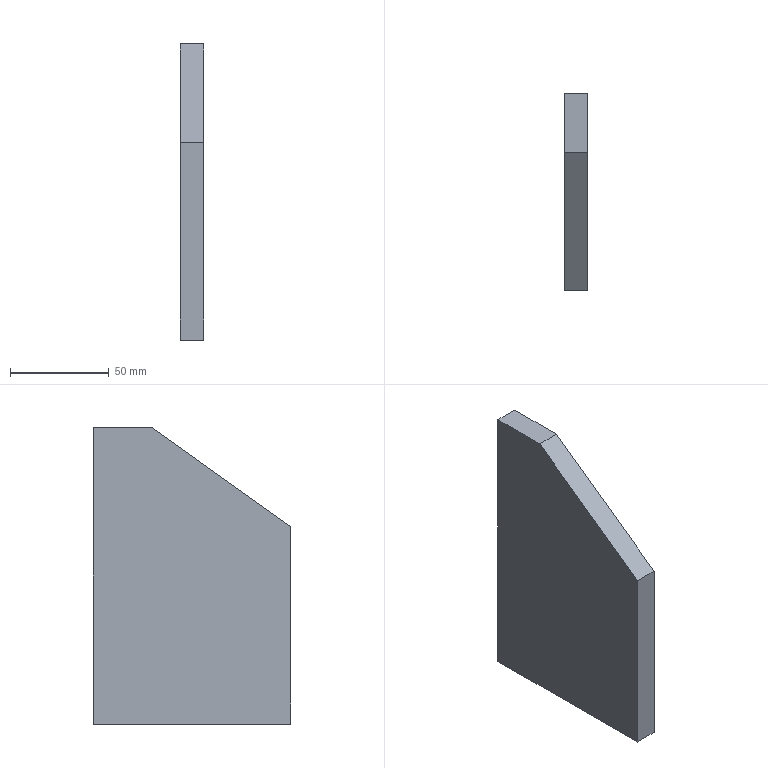Component | SolidWorks | 8TC-A15004-80-04A-1 | 1 solid | 27 faces | box 12 x 100 x 150 mm | volume 156512 mm3 | cylinder 10 | cone 10 | plane 7 | commonest cylinder face diameters 6 x10 | material A3
build123d program:
from build123d import *

# Parameters (mm, degrees)
BOSS_EXTRUDE1_DEPTH   = 6
M6_TAPPED_HOLE1_D     = 6
M6_TAPPED_HOLE1_DEPTH = 17
M6_TAPPED_HOLE1_TIP   = 1.803
M6_TAPPED_HOLE2_D     = 6
M6_TAPPED_HOLE2_DEPTH = 17
M6_TAPPED_HOLE2_TIP   = 1.803


with BuildPart() as part:
    # Sketch1 → Boss-Extrude1 (new, symmetric)
    with BuildSketch(Plane(origin=(0, 0, 0), x_dir=(1, 0, 0), z_dir=(0, 1, 0))):
        Polygon((0, 0), (0, 150), (30, 150), (100, 100), (100, 0), align=None)
    extrude(amount=BOSS_EXTRUDE1_DEPTH, both=True)

    # M6 Tapped Hole1
    with Locations(Plane.ZY):
        with Locations((-30, 0), (-80, 0), (-130, 0)):
            Hole(M6_TAPPED_HOLE1_D / 2, depth=M6_TAPPED_HOLE1_DEPTH)
            with Locations((0, 0, -(M6_TAPPED_HOLE1_DEPTH + M6_TAPPED_HOLE1_TIP / 2))):  # 118° drill point
                Cone(0, M6_TAPPED_HOLE1_D / 2, M6_TAPPED_HOLE1_TIP, mode=Mode.SUBTRACT)

    # M6 Tapped Hole2
    with Locations(Plane.XY):
        with Locations((20, 0), (80, 0)):
            Hole(M6_TAPPED_HOLE2_D / 2, depth=M6_TAPPED_HOLE2_DEPTH)
            with Locations((0, 0, -(M6_TAPPED_HOLE2_DEPTH + M6_TAPPED_HOLE2_TIP / 2))):  # 118° drill point
                Cone(0, M6_TAPPED_HOLE2_D / 2, M6_TAPPED_HOLE2_TIP, mode=Mode.SUBTRACT)


solid = part.part

# Placed as in the assembly
solid = solid.moved(Location((16, -7.5, 40), (180, 0, 90)))
STEP:
#1=COLOUR_RGB('',0.7922,0.8196,0.9333);
#2=FILL_AREA_STYLE_COLOUR('',#1);
#3=FILL_AREA_STYLE('',(#2));
#4=SURFACE_STYLE_FILL_AREA(#3);
#5=SURFACE_SIDE_STYLE('',(#4));
#6=SURFACE_STYLE_USAGE(.BOTH.,#5);
#7=PRESENTATION_STYLE_ASSIGNMENT((#6));
#8=CARTESIAN_POINT('',(0.6299,-0.9646,2.244));
#9=VERTEX_POINT('',#8);
#10=CARTESIAN_POINT('',(0.6299,-1.201,2.244));
#11=VERTEX_POINT('',#10);
#12=CARTESIAN_POINT('',(0.6299,-1.083,2.244));
#13=DIRECTION('',(0.,0.,-1.));
#14=DIRECTION('',(0.,-1.,0.));
#15=AXIS2_PLACEMENT_3D('',#12,#13,#14);
#16=CIRCLE('',#15,0.1181);
#17=EDGE_CURVE('',#9,#11,#16,.T.);
#18=ORIENTED_EDGE('',*,*,#17,.F.);
#19=CARTESIAN_POINT('',(0.6299,-0.9646,1.575));
#20=VERTEX_POINT('',#19);
#21=CARTESIAN_POINT('',(0.6299,-0.9646,1.575));
#22=DIRECTION('',(0.,0.,-1.));
#23=VECTOR('',#22,39.37);
#24=LINE('',#21,#23);
#25=EDGE_CURVE('',#9,#20,#24,.T.);
#26=ORIENTED_EDGE('',*,*,#25,.T.);
#27=CARTESIAN_POINT('',(0.6299,-1.201,1.575));
#28=VERTEX_POINT('',#27);
#29=CARTESIAN_POINT('',(0.6299,-1.083,1.575));
#30=DIRECTION('',(0.,0.,-1.));
#31=DIRECTION('',(0.,-1.,0.));
#32=AXIS2_PLACEMENT_3D('',#29,#30,#31);
#33=CIRCLE('',#32,0.1181);
#34=EDGE_CURVE('',#20,#28,#33,.T.);
#35=ORIENTED_EDGE('',*,*,#34,.T.);
#36=CARTESIAN_POINT('',(0.6299,-1.201,1.575));
#37=DIRECTION('',(0.,0.,-1.));
#38=VECTOR('',#37,39.37);
#39=LINE('',#36,#38);
#40=EDGE_CURVE('',#11,#28,#39,.T.);
#41=ORIENTED_EDGE('',*,*,#40,.F.);
#42=EDGE_LOOP('',(#18,#26,#35,#41));
#43=FACE_OUTER_BOUND('',#42,.T.);
#44=CARTESIAN_POINT('',(0.6299,-1.083,1.575));
#45=DIRECTION('',(0.,0.,-1.));
#46=DIRECTION('',(0.,-1.,0.));
#47=AXIS2_PLACEMENT_3D('',#44,#45,#46);
#48=CYLINDRICAL_SURFACE('',#47,0.1181);
#49=ADVANCED_FACE('',(#43),#48,.F.);
#50=CARTESIAN_POINT('',(0.6299,-1.083,2.315));
#51=VERTEX_POINT('',#50);
#52=CARTESIAN_POINT('',(0.6299,-1.201,2.244));
#53=DIRECTION('',(0.,-0.8572,-0.515));
#54=VECTOR('',#53,39.37);
#55=LINE('',#52,#54);
#56=EDGE_CURVE('',#51,#11,#55,.T.);
#57=ORIENTED_EDGE('',*,*,#56,.F.);
#58=CARTESIAN_POINT('',(0.6299,-0.9646,2.244));
#59=DIRECTION('',(-0.,0.8572,-0.515));
#60=VECTOR('',#59,39.37);
#61=LINE('',#58,#60);
#62=EDGE_CURVE('',#51,#9,#61,.T.);
#63=ORIENTED_EDGE('',*,*,#62,.T.);
#64=ORIENTED_EDGE('',*,*,#17,.T.);
#65=EDGE_LOOP('',(#57,#63,#64));
#66=FACE_OUTER_BOUND('',#65,.T.);
#67=CARTESIAN_POINT('',(0.6299,-1.083,2.244));
#68=DIRECTION('',(0.,0.,-1.));
#69=DIRECTION('',(0.,-1.,0.));
#70=AXIS2_PLACEMENT_3D('',#67,#68,#69);
#71=CONICAL_SURFACE('',#70,0.1181,1.03);
#72=ADVANCED_FACE('',(#66),#71,.F.);
#73=CARTESIAN_POINT('',(0.6299,-3.327,2.244));
#74=VERTEX_POINT('',#73);
#75=CARTESIAN_POINT('',(0.6299,-3.563,2.244));
#76=VERTEX_POINT('',#75);
#77=CARTESIAN_POINT('',(0.6299,-3.445,2.244));
#78=DIRECTION('',(0.,0.,-1.));
#79=DIRECTION('',(0.,-1.,0.));
#80=AXIS2_PLACEMENT_3D('',#77,#78,#79);
#81=CIRCLE('',#80,0.1181);
#82=EDGE_CURVE('',#74,#76,#81,.T.);
#83=ORIENTED_EDGE('',*,*,#82,.F.);
#84=CARTESIAN_POINT('',(0.6299,-3.327,1.575));
#85=VERTEX_POINT('',#84);
#86=CARTESIAN_POINT('',(0.6299,-3.327,1.575));
#87=DIRECTION('',(0.,0.,-1.));
#88=VECTOR('',#87,39.37);
#89=LINE('',#86,#88);
#90=EDGE_CURVE('',#74,#85,#89,.T.);
#91=ORIENTED_EDGE('',*,*,#90,.T.);
#92=CARTESIAN_POINT('',(0.6299,-3.563,1.575));
#93=VERTEX_POINT('',#92);
#94=CARTESIAN_POINT('',(0.6299,-3.445,1.575));
#95=DIRECTION('',(0.,0.,-1.));
#96=DIRECTION('',(0.,-1.,0.));
#97=AXIS2_PLACEMENT_3D('',#94,#95,#96);
#98=CIRCLE('',#97,0.1181);
#99=EDGE_CURVE('',#85,#93,#98,.T.);
#100=ORIENTED_EDGE('',*,*,#99,.T.);
#101=CARTESIAN_POINT('',(0.6299,-3.563,1.575));
#102=DIRECTION('',(0.,0.,-1.));
#103=VECTOR('',#102,39.37);
#104=LINE('',#101,#103);
#105=EDGE_CURVE('',#76,#93,#104,.T.);
#106=ORIENTED_EDGE('',*,*,#105,.F.);
#107=EDGE_LOOP('',(#83,#91,#100,#106));
#108=FACE_OUTER_BOUND('',#107,.T.);
#109=CARTESIAN_POINT('',(0.6299,-3.445,1.575));
#110=DIRECTION('',(0.,0.,-1.));
#111=DIRECTION('',(0.,-1.,0.));
#112=AXIS2_PLACEMENT_3D('',#109,#110,#111);
#113=CYLINDRICAL_SURFACE('',#112,0.1181);
#114=ADVANCED_FACE('',(#108),#113,.F.);
#115=CARTESIAN_POINT('',(0.6299,-3.445,2.315));
#116=VERTEX_POINT('',#115);
#117=CARTESIAN_POINT('',(0.6299,-3.563,2.244));
#118=DIRECTION('',(0.,-0.8572,-0.515));
#119=VECTOR('',#118,39.37);
#120=LINE('',#117,#119);
#121=EDGE_CURVE('',#116,#76,#120,.T.);
#122=ORIENTED_EDGE('',*,*,#121,.F.);
#123=CARTESIAN_POINT('',(0.6299,-3.327,2.244));
#124=DIRECTION('',(-0.,0.8572,-0.515));
#125=VECTOR('',#124,39.37);
#126=LINE('',#123,#125);
#127=EDGE_CURVE('',#116,#74,#126,.T.);
#128=ORIENTED_EDGE('',*,*,#127,.T.);
#129=ORIENTED_EDGE('',*,*,#82,.T.);
#130=EDGE_LOOP('',(#122,#128,#129));
#131=FACE_OUTER_BOUND('',#130,.T.);
#132=CARTESIAN_POINT('',(0.6299,-3.445,2.244));
#133=DIRECTION('',(0.,0.,-1.));
#134=DIRECTION('',(0.,-1.,0.));
#135=AXIS2_PLACEMENT_3D('',#132,#133,#134);
#136=CONICAL_SURFACE('',#135,0.1181,1.03);
#137=ADVANCED_FACE('',(#131),#136,.F.);
#138=CARTESIAN_POINT('',(0.6299,-0.9646,2.874));
#139=VERTEX_POINT('',#138);
#140=CARTESIAN_POINT('',(0.6299,-0.9646,2.638));
#141=VERTEX_POINT('',#140);
#142=CARTESIAN_POINT('',(0.6299,-0.9646,2.756));
#143=DIRECTION('',(-0.,1.,0.));
#144=DIRECTION('',(0.,0.,-1.));
#145=AXIS2_PLACEMENT_3D('',#142,#143,#144);
#146=CIRCLE('',#145,0.1181);
#147=EDGE_CURVE('',#139,#141,#146,.T.);
#148=ORIENTED_EDGE('',*,*,#147,.F.);
#149=CARTESIAN_POINT('',(0.6299,-0.2953,2.874));
#150=VERTEX_POINT('',#149);
#151=CARTESIAN_POINT('',(0.6299,-0.2953,2.874));
#152=DIRECTION('',(-0.,1.,0.));
#153=VECTOR('',#152,39.37);
#154=LINE('',#151,#153);
#155=EDGE_CURVE('',#139,#150,#154,.T.);
#156=ORIENTED_EDGE('',*,*,#155,.T.);
#157=CARTESIAN_POINT('',(0.6299,-0.2953,2.638));
#158=VERTEX_POINT('',#157);
#159=CARTESIAN_POINT('',(0.6299,-0.2953,2.756));
#160=DIRECTION('',(-0.,1.,0.));
#161=DIRECTION('',(0.,0.,-1.));
#162=AXIS2_PLACEMENT_3D('',#159,#160,#161);
#163=CIRCLE('',#162,0.1181);
#164=EDGE_CURVE('',#150,#158,#163,.T.);
#165=ORIENTED_EDGE('',*,*,#164,.T.);
#166=CARTESIAN_POINT('',(0.6299,-0.2953,2.638));
#167=DIRECTION('',(-0.,1.,0.));
#168=VECTOR('',#167,39.37);
#169=LINE('',#166,#168);
#170=EDGE_CURVE('',#141,#158,#169,.T.);
#171=ORIENTED_EDGE('',*,*,#170,.F.);
#172=EDGE_LOOP('',(#148,#156,#165,#171));
#173=FACE_OUTER_BOUND('',#172,.T.);
#174=CARTESIAN_POINT('',(0.6299,-0.2953,2.756));
#175=DIRECTION('',(-0.,1.,0.));
#176=DIRECTION('',(0.,0.,-1.));
#177=AXIS2_PLACEMENT_3D('',#174,#175,#176);
#178=CYLINDRICAL_SURFACE('',#177,0.1181);
#179=ADVANCED_FACE('',(#173),#178,.F.);
#180=CARTESIAN_POINT('',(0.6299,-1.036,2.756));
#181=VERTEX_POINT('',#180);
#182=CARTESIAN_POINT('',(0.6299,-0.9646,2.638));
#183=DIRECTION('',(-0.,0.515,-0.8572));
#184=VECTOR('',#183,39.37);
#185=LINE('',#182,#184);
#186=EDGE_CURVE('',#181,#141,#185,.T.);
#187=ORIENTED_EDGE('',*,*,#186,.F.);
#188=CARTESIAN_POINT('',(0.6299,-0.9646,2.874));
#189=DIRECTION('',(-0.,0.515,0.8572));
#190=VECTOR('',#189,39.37);
#191=LINE('',#188,#190);
#192=EDGE_CURVE('',#181,#139,#191,.T.);
#193=ORIENTED_EDGE('',*,*,#192,.T.);
#194=ORIENTED_EDGE('',*,*,#147,.T.);
#195=EDGE_LOOP('',(#187,#193,#194));
#196=FACE_OUTER_BOUND('',#195,.T.);
#197=CARTESIAN_POINT('',(0.6299,-0.9646,2.756));
#198=DIRECTION('',(-0.,1.,0.));
#199=DIRECTION('',(0.,0.,-1.));
#200=AXIS2_PLACEMENT_3D('',#197,#198,#199);
#201=CONICAL_SURFACE('',#200,0.1181,1.03);
#202=ADVANCED_FACE('',(#196),#201,.F.);
#203=CARTESIAN_POINT('',(0.6299,-0.9646,4.843));
#204=VERTEX_POINT('',#203);
#205=CARTESIAN_POINT('',(0.6299,-0.9646,4.606));
#206=VERTEX_POINT('',#205);
#207=CARTESIAN_POINT('',(0.6299,-0.9646,4.724));
#208=DIRECTION('',(-0.,1.,0.));
#209=DIRECTION('',(0.,0.,-1.));
#210=AXIS2_PLACEMENT_3D('',#207,#208,#209);
#211=CIRCLE('',#210,0.1181);
#212=EDGE_CURVE('',#204,#206,#211,.T.);
#213=ORIENTED_EDGE('',*,*,#212,.F.);
#214=CARTESIAN_POINT('',(0.6299,-0.2953,4.843));
#215=VERTEX_POINT('',#214);
#216=CARTESIAN_POINT('',(0.6299,-0.2953,4.843));
#217=DIRECTION('',(-0.,1.,0.));
#218=VECTOR('',#217,39.37);
#219=LINE('',#216,#218);
#220=EDGE_CURVE('',#204,#215,#219,.T.);
#221=ORIENTED_EDGE('',*,*,#220,.T.);
#222=CARTESIAN_POINT('',(0.6299,-0.2953,4.606));
#223=VERTEX_POINT('',#222);
#224=CARTESIAN_POINT('',(0.6299,-0.2953,4.724));
#225=DIRECTION('',(-0.,1.,0.));
#226=DIRECTION('',(0.,0.,-1.));
#227=AXIS2_PLACEMENT_3D('',#224,#225,#226);
#228=CIRCLE('',#227,0.1181);
#229=EDGE_CURVE('',#215,#223,#228,.T.);
#230=ORIENTED_EDGE('',*,*,#229,.T.);
#231=CARTESIAN_POINT('',(0.6299,-0.2953,4.606));
#232=DIRECTION('',(-0.,1.,0.));
#233=VECTOR('',#232,39.37);
#234=LINE('',#231,#233);
#235=EDGE_CURVE('',#206,#223,#234,.T.);
#236=ORIENTED_EDGE('',*,*,#235,.F.);
#237=EDGE_LOOP('',(#213,#221,#230,#236));
#238=FACE_OUTER_BOUND('',#237,.T.);
#239=CARTESIAN_POINT('',(0.6299,-0.2953,4.724));
#240=DIRECTION('',(-0.,1.,0.));
#241=DIRECTION('',(0.,0.,-1.));
#242=AXIS2_PLACEMENT_3D('',#239,#240,#241);
#243=CYLINDRICAL_SURFACE('',#242,0.1181);
#244=ADVANCED_FACE('',(#238),#243,.F.);
#245=CARTESIAN_POINT('',(0.6299,-1.036,4.724));
#246=VERTEX_POINT('',#245);
#247=CARTESIAN_POINT('',(0.6299,-0.9646,4.606));
#248=DIRECTION('',(-0.,0.515,-0.8572));
#249=VECTOR('',#248,39.37);
#250=LINE('',#247,#249);
#251=EDGE_CURVE('',#246,#206,#250,.T.);
#252=ORIENTED_EDGE('',*,*,#251,.F.);
#253=CARTESIAN_POINT('',(0.6299,-0.9646,4.843));
#254=DIRECTION('',(-0.,0.515,0.8572));
#255=VECTOR('',#254,39.37);
#256=LINE('',#253,#255);
#257=EDGE_CURVE('',#246,#204,#256,.T.);
#258=ORIENTED_EDGE('',*,*,#257,.T.);
#259=ORIENTED_EDGE('',*,*,#212,.T.);
#260=EDGE_LOOP('',(#252,#258,#259));
#261=FACE_OUTER_BOUND('',#260,.T.);
#262=CARTESIAN_POINT('',(0.6299,-0.9646,4.724));
#263=DIRECTION('',(-0.,1.,0.));
#264=DIRECTION('',(0.,0.,-1.));
#265=AXIS2_PLACEMENT_3D('',#262,#263,#264);
#266=CONICAL_SURFACE('',#265,0.1181,1.03);
#267=ADVANCED_FACE('',(#261),#266,.F.);
#268=CARTESIAN_POINT('',(0.6299,-0.9646,6.811));
#269=VERTEX_POINT('',#268);
#270=CARTESIAN_POINT('',(0.6299,-0.9646,6.575));
#271=VERTEX_POINT('',#270);
#272=CARTESIAN_POINT('',(0.6299,-0.9646,6.693));
#273=DIRECTION('',(-0.,1.,0.));
#274=DIRECTION('',(0.,0.,-1.));
#275=AXIS2_PLACEMENT_3D('',#272,#273,#274);
#276=CIRCLE('',#275,0.1181);
#277=EDGE_CURVE('',#269,#271,#276,.T.);
#278=ORIENTED_EDGE('',*,*,#277,.F.);
#279=CARTESIAN_POINT('',(0.6299,-0.2953,6.811));
#280=VERTEX_POINT('',#279);
#281=CARTESIAN_POINT('',(0.6299,-0.2953,6.811));
#282=DIRECTION('',(-0.,1.,0.));
#283=VECTOR('',#282,39.37);
#284=LINE('',#281,#283);
#285=EDGE_CURVE('',#269,#280,#284,.T.);
#286=ORIENTED_EDGE('',*,*,#285,.T.);
#287=CARTESIAN_POINT('',(0.6299,-0.2953,6.575));
#288=VERTEX_POINT('',#287);
#289=CARTESIAN_POINT('',(0.6299,-0.2953,6.693));
#290=DIRECTION('',(-0.,1.,0.));
#291=DIRECTION('',(0.,0.,-1.));
#292=AXIS2_PLACEMENT_3D('',#289,#290,#291);
#293=CIRCLE('',#292,0.1181);
#294=EDGE_CURVE('',#280,#288,#293,.T.);
#295=ORIENTED_EDGE('',*,*,#294,.T.);
#296=CARTESIAN_POINT('',(0.6299,-0.2953,6.575));
#297=DIRECTION('',(-0.,1.,0.));
#298=VECTOR('',#297,39.37);
#299=LINE('',#296,#298);
#300=EDGE_CURVE('',#271,#288,#299,.T.);
#301=ORIENTED_EDGE('',*,*,#300,.F.);
#302=EDGE_LOOP('',(#278,#286,#295,#301));
#303=FACE_OUTER_BOUND('',#302,.T.);
#304=CARTESIAN_POINT('',(0.6299,-0.2953,6.693));
#305=DIRECTION('',(-0.,1.,0.));
#306=DIRECTION('',(0.,0.,-1.));
#307=AXIS2_PLACEMENT_3D('',#304,#305,#306);
#308=CYLINDRICAL_SURFACE('',#307,0.1181);
#309=ADVANCED_FACE('',(#303),#308,.F.);
#310=CARTESIAN_POINT('',(0.6299,-1.036,6.693));
#311=VERTEX_POINT('',#310);
#312=CARTESIAN_POINT('',(0.6299,-0.9646,6.575));
#313=DIRECTION('',(-0.,0.515,-0.8572));
#314=VECTOR('',#313,39.37);
#315=LINE('',#312,#314);
#316=EDGE_CURVE('',#311,#271,#315,.T.);
#317=ORIENTED_EDGE('',*,*,#316,.F.);
#318=CARTESIAN_POINT('',(0.6299,-0.9646,6.811));
#319=DIRECTION('',(-0.,0.515,0.8572));
#320=VECTOR('',#319,39.37);
#321=LINE('',#318,#320);
#322=EDGE_CURVE('',#311,#269,#321,.T.);
#323=ORIENTED_EDGE('',*,*,#322,.T.);
#324=ORIENTED_EDGE('',*,*,#277,.T.);
#325=EDGE_LOOP('',(#317,#323,#324));
#326=FACE_OUTER_BOUND('',#325,.T.);
#327=CARTESIAN_POINT('',(0.6299,-0.9646,6.693));
#328=DIRECTION('',(-0.,1.,0.));
#329=DIRECTION('',(0.,0.,-1.));
#330=AXIS2_PLACEMENT_3D('',#327,#328,#329);
#331=CONICAL_SURFACE('',#330,0.1181,1.03);
#332=ADVANCED_FACE('',(#326),#331,.F.);
#333=CARTESIAN_POINT('',(0.6299,-0.2953,2.756));
#334=DIRECTION('',(-0.,1.,0.));
#335=DIRECTION('',(0.,0.,-1.));
#336=AXIS2_PLACEMENT_3D('',#333,#334,#335);
#337=CIRCLE('',#336,0.1181);
#338=EDGE_CURVE('',#158,#150,#337,.T.);
#339=ORIENTED_EDGE('',*,*,#338,.F.);
#340=ORIENTED_EDGE('',*,*,#164,.F.);
#341=EDGE_LOOP('',(#339,#340));
#342=FACE_BOUND('',#341,.T.);
#343=CARTESIAN_POINT('',(0.6299,-0.2953,6.693));
#344=DIRECTION('',(-0.,1.,0.));
#345=DIRECTION('',(0.,0.,-1.));
#346=AXIS2_PLACEMENT_3D('',#343,#344,#345);
#347=CIRCLE('',#346,0.1181);
#348=EDGE_CURVE('',#288,#280,#347,.T.);
#349=ORIENTED_EDGE('',*,*,#348,.F.);
#350=ORIENTED_EDGE('',*,*,#294,.F.);
#351=EDGE_LOOP('',(#349,#350));
#352=FACE_BOUND('',#351,.T.);
#353=CARTESIAN_POINT('',(0.8661,-0.2953,7.48));
#354=VERTEX_POINT('',#353);
#355=CARTESIAN_POINT('',(0.8661,-0.2953,1.575));
#356=VERTEX_POINT('',#355);
#357=CARTESIAN_POINT('',(0.8661,-0.2953,1.575));
#358=DIRECTION('',(0.,0.,-1.));
#359=VECTOR('',#358,39.37);
#360=LINE('',#357,#359);
#361=EDGE_CURVE('',#354,#356,#360,.T.);
#362=ORIENTED_EDGE('',*,*,#361,.T.);
#363=CARTESIAN_POINT('',(0.3937,-0.2953,1.575));
#364=VERTEX_POINT('',#363);
#365=CARTESIAN_POINT('',(0.3937,-0.2953,1.575));
#366=DIRECTION('',(1.,0.,0.));
#367=VECTOR('',#366,39.37);
#368=LINE('',#365,#367);
#369=EDGE_CURVE('',#364,#356,#368,.T.);
#370=ORIENTED_EDGE('',*,*,#369,.F.);
#371=CARTESIAN_POINT('',(0.3937,-0.2953,7.48));
#372=VERTEX_POINT('',#371);
#373=CARTESIAN_POINT('',(0.3937,-0.2953,1.575));
#374=DIRECTION('',(0.,0.,-1.));
#375=VECTOR('',#374,39.37);
#376=LINE('',#373,#375);
#377=EDGE_CURVE('',#372,#364,#376,.T.);
#378=ORIENTED_EDGE('',*,*,#377,.F.);
#379=CARTESIAN_POINT('',(0.3937,-0.2953,7.48));
#380=DIRECTION('',(1.,0.,0.));
#381=VECTOR('',#380,39.37);
#382=LINE('',#379,#381);
#383=EDGE_CURVE('',#372,#354,#382,.T.);
#384=ORIENTED_EDGE('',*,*,#383,.T.);
#385=EDGE_LOOP('',(#362,#370,#378,#384));
#386=FACE_OUTER_BOUND('',#385,.T.);
#387=CARTESIAN_POINT('',(0.6299,-0.2953,4.724));
#388=DIRECTION('',(-0.,1.,0.));
#389=DIRECTION('',(0.,0.,-1.));
#390=AXIS2_PLACEMENT_3D('',#387,#388,#389);
#391=CIRCLE('',#390,0.1181);
#392=EDGE_CURVE('',#223,#215,#391,.T.);
#393=ORIENTED_EDGE('',*,*,#392,.F.);
#394=ORIENTED_EDGE('',*,*,#229,.F.);
#395=EDGE_LOOP('',(#393,#394));
#396=FACE_BOUND('',#395,.T.);
#397=CARTESIAN_POINT('',(0.3937,-0.2953,1.575));
#398=DIRECTION('',(0.,-1.,0.));
#399=DIRECTION('',(0.,0.,1.));
#400=AXIS2_PLACEMENT_3D('',#397,#398,#399);
#401=PLANE('',#400);
#402=ADVANCED_FACE('',(#342,#352,#386,#396),#401,.F.);
#403=CARTESIAN_POINT('',(0.6299,-1.083,1.575));
#404=DIRECTION('',(0.,0.,-1.));
#405=DIRECTION('',(0.,-1.,0.));
#406=AXIS2_PLACEMENT_3D('',#403,#404,#405);
#407=CIRCLE('',#406,0.1181);
#408=EDGE_CURVE('',#28,#20,#407,.T.);
#409=ORIENTED_EDGE('',*,*,#408,.F.);
#410=ORIENTED_EDGE('',*,*,#34,.F.);
#411=EDGE_LOOP('',(#409,#410));
#412=FACE_BOUND('',#411,.T.);
#413=CARTESIAN_POINT('',(0.6299,-3.445,1.575));
#414=DIRECTION('',(0.,0.,-1.));
#415=DIRECTION('',(0.,-1.,0.));
#416=AXIS2_PLACEMENT_3D('',#413,#414,#415);
#417=CIRCLE('',#416,0.1181);
#418=EDGE_CURVE('',#93,#85,#417,.T.);
#419=ORIENTED_EDGE('',*,*,#418,.F.);
#420=ORIENTED_EDGE('',*,*,#99,.F.);
#421=EDGE_LOOP('',(#419,#420));
#422=FACE_BOUND('',#421,.T.);
#423=CARTESIAN_POINT('',(0.8661,-4.232,1.575));
#424=VERTEX_POINT('',#423);
#425=CARTESIAN_POINT('',(0.8661,-4.232,1.575));
#426=DIRECTION('',(0.,-1.,0.));
#427=VECTOR('',#426,39.37);
#428=LINE('',#425,#427);
#429=EDGE_CURVE('',#356,#424,#428,.T.);
#430=ORIENTED_EDGE('',*,*,#429,.T.);
#431=CARTESIAN_POINT('',(0.3937,-4.232,1.575));
#432=VERTEX_POINT('',#431);
#433=CARTESIAN_POINT('',(0.3937,-4.232,1.575));
#434=DIRECTION('',(1.,0.,0.));
#435=VECTOR('',#434,39.37);
#436=LINE('',#433,#435);
#437=EDGE_CURVE('',#432,#424,#436,.T.);
#438=ORIENTED_EDGE('',*,*,#437,.F.);
#439=CARTESIAN_POINT('',(0.3937,-4.232,1.575));
#440=DIRECTION('',(0.,-1.,0.));
#441=VECTOR('',#440,39.37);
#442=LINE('',#439,#441);
#443=EDGE_CURVE('',#364,#432,#442,.T.);
#444=ORIENTED_EDGE('',*,*,#443,.F.);
#445=ORIENTED_EDGE('',*,*,#369,.T.);
#446=EDGE_LOOP('',(#430,#438,#444,#445));
#447=FACE_OUTER_BOUND('',#446,.T.);
#448=CARTESIAN_POINT('',(0.3937,-4.232,1.575));
#449=DIRECTION('',(0.,0.,1.));
#450=DIRECTION('',(-0.,1.,0.));
#451=AXIS2_PLACEMENT_3D('',#448,#449,#450);
#452=PLANE('',#451);
#453=ADVANCED_FACE('',(#412,#422,#447),#452,.F.);
#454=CARTESIAN_POINT('',(0.8661,-4.232,5.512));
#455=VERTEX_POINT('',#454);
#456=CARTESIAN_POINT('',(0.8661,-4.232,5.512));
#457=DIRECTION('',(-0.,0.,1.));
#458=VECTOR('',#457,39.37);
#459=LINE('',#456,#458);
#460=EDGE_CURVE('',#424,#455,#459,.T.);
#461=ORIENTED_EDGE('',*,*,#460,.T.);
#462=CARTESIAN_POINT('',(0.3937,-4.232,5.512));
#463=VERTEX_POINT('',#462);
#464=CARTESIAN_POINT('',(0.3937,-4.232,5.512));
#465=DIRECTION('',(1.,0.,0.));
#466=VECTOR('',#465,39.37);
#467=LINE('',#464,#466);
#468=EDGE_CURVE('',#463,#455,#467,.T.);
#469=ORIENTED_EDGE('',*,*,#468,.F.);
#470=CARTESIAN_POINT('',(0.3937,-4.232,5.512));
#471=DIRECTION('',(-0.,0.,1.));
#472=VECTOR('',#471,39.37);
#473=LINE('',#470,#472);
#474=EDGE_CURVE('',#432,#463,#473,.T.);
#475=ORIENTED_EDGE('',*,*,#474,.F.);
#476=ORIENTED_EDGE('',*,*,#437,.T.);
#477=EDGE_LOOP('',(#461,#469,#475,#476));
#478=FACE_OUTER_BOUND('',#477,.T.);
#479=CARTESIAN_POINT('',(0.3937,-4.232,5.512));
#480=DIRECTION('',(-0.,1.,-0.));
#481=DIRECTION('',(0.,-0.,-1.));
#482=AXIS2_PLACEMENT_3D('',#479,#480,#481);
#483=PLANE('',#482);
#484=ADVANCED_FACE('',(#478),#483,.F.);
#485=CARTESIAN_POINT('',(0.8661,-1.476,7.48));
#486=VERTEX_POINT('',#485);
#487=CARTESIAN_POINT('',(0.8661,-1.476,7.48));
#488=DIRECTION('',(-0.,0.8137,0.5812));
#489=VECTOR('',#488,39.37);
#490=LINE('',#487,#489);
#491=EDGE_CURVE('',#455,#486,#490,.T.);
#492=ORIENTED_EDGE('',*,*,#491,.T.);
#493=CARTESIAN_POINT('',(0.3937,-1.476,7.48));
#494=VERTEX_POINT('',#493);
#495=CARTESIAN_POINT('',(0.3937,-1.476,7.48));
#496=DIRECTION('',(1.,0.,0.));
#497=VECTOR('',#496,39.37);
#498=LINE('',#495,#497);
#499=EDGE_CURVE('',#494,#486,#498,.T.);
#500=ORIENTED_EDGE('',*,*,#499,.F.);
#501=CARTESIAN_POINT('',(0.3937,-1.476,7.48));
#502=DIRECTION('',(-0.,0.8137,0.5812));
#503=VECTOR('',#502,39.37);
#504=LINE('',#501,#503);
#505=EDGE_CURVE('',#463,#494,#504,.T.);
#506=ORIENTED_EDGE('',*,*,#505,.F.);
#507=ORIENTED_EDGE('',*,*,#468,.T.);
#508=EDGE_LOOP('',(#492,#500,#506,#507));
#509=FACE_OUTER_BOUND('',#508,.T.);
#510=CARTESIAN_POINT('',(0.3937,-1.476,7.48));
#511=DIRECTION('',(-0.,0.5812,-0.8137));
#512=DIRECTION('',(0.,-0.8137,-0.5812));
#513=AXIS2_PLACEMENT_3D('',#510,#511,#512);
#514=PLANE('',#513);
#515=ADVANCED_FACE('',(#509),#514,.F.);
#516=CARTESIAN_POINT('',(0.8661,-0.2953,7.48));
#517=DIRECTION('',(-0.,1.,0.));
#518=VECTOR('',#517,39.37);
#519=LINE('',#516,#518);
#520=EDGE_CURVE('',#486,#354,#519,.T.);
#521=ORIENTED_EDGE('',*,*,#520,.T.);
#522=ORIENTED_EDGE('',*,*,#383,.F.);
#523=CARTESIAN_POINT('',(0.3937,-0.2953,7.48));
#524=DIRECTION('',(-0.,1.,0.));
#525=VECTOR('',#524,39.37);
#526=LINE('',#523,#525);
#527=EDGE_CURVE('',#494,#372,#526,.T.);
#528=ORIENTED_EDGE('',*,*,#527,.F.);
#529=ORIENTED_EDGE('',*,*,#499,.T.);
#530=EDGE_LOOP('',(#521,#522,#528,#529));
#531=FACE_OUTER_BOUND('',#530,.T.);
#532=CARTESIAN_POINT('',(0.3937,-0.2953,7.48));
#533=DIRECTION('',(0.,0.,-1.));
#534=DIRECTION('',(0.,-1.,0.));
#535=AXIS2_PLACEMENT_3D('',#532,#533,#534);
#536=PLANE('',#535);
#537=ADVANCED_FACE('',(#531),#536,.F.);
#538=ORIENTED_EDGE('',*,*,#443,.T.);
#539=ORIENTED_EDGE('',*,*,#474,.T.);
#540=ORIENTED_EDGE('',*,*,#505,.T.);
#541=ORIENTED_EDGE('',*,*,#527,.T.);
#542=ORIENTED_EDGE('',*,*,#377,.T.);
#543=EDGE_LOOP('',(#538,#539,#540,#541,#542));
#544=FACE_OUTER_BOUND('',#543,.T.);
#545=CARTESIAN_POINT('',(0.3937,-0.2953,1.575));
#546=DIRECTION('',(1.,0.,0.));
#547=DIRECTION('',(0.,0.,1.));
#548=AXIS2_PLACEMENT_3D('',#545,#546,#547);
#549=PLANE('',#548);
#550=ADVANCED_FACE('',(#544),#549,.F.);
#551=ORIENTED_EDGE('',*,*,#429,.F.);
#552=ORIENTED_EDGE('',*,*,#361,.F.);
#553=ORIENTED_EDGE('',*,*,#520,.F.);
#554=ORIENTED_EDGE('',*,*,#491,.F.);
#555=ORIENTED_EDGE('',*,*,#460,.F.);
#556=EDGE_LOOP('',(#551,#552,#553,#554,#555));
#557=FACE_OUTER_BOUND('',#556,.T.);
#558=CARTESIAN_POINT('',(0.8661,-0.2953,1.575));
#559=DIRECTION('',(1.,0.,0.));
#560=DIRECTION('',(0.,0.,1.));
#561=AXIS2_PLACEMENT_3D('',#558,#559,#560);
#562=PLANE('',#561);
#563=ADVANCED_FACE('',(#557),#562,.T.);
#564=ORIENTED_EDGE('',*,*,#322,.F.);
#565=ORIENTED_EDGE('',*,*,#316,.T.);
#566=CARTESIAN_POINT('',(0.6299,-0.9646,6.693));
#567=DIRECTION('',(-0.,1.,0.));
#568=DIRECTION('',(0.,0.,-1.));
#569=AXIS2_PLACEMENT_3D('',#566,#567,#568);
#570=CIRCLE('',#569,0.1181);
#571=EDGE_CURVE('',#271,#269,#570,.T.);
#572=ORIENTED_EDGE('',*,*,#571,.T.);
#573=EDGE_LOOP('',(#564,#565,#572));
#574=FACE_OUTER_BOUND('',#573,.T.);
#575=CARTESIAN_POINT('',(0.6299,-0.9646,6.693));
#576=DIRECTION('',(-0.,1.,0.));
#577=DIRECTION('',(0.,0.,-1.));
#578=AXIS2_PLACEMENT_3D('',#575,#576,#577);
#579=CONICAL_SURFACE('',#578,0.1181,1.03);
#580=ADVANCED_FACE('',(#574),#579,.F.);
#581=ORIENTED_EDGE('',*,*,#285,.F.);
#582=ORIENTED_EDGE('',*,*,#571,.F.);
#583=ORIENTED_EDGE('',*,*,#300,.T.);
#584=ORIENTED_EDGE('',*,*,#348,.T.);
#585=EDGE_LOOP('',(#581,#582,#583,#584));
#586=FACE_OUTER_BOUND('',#585,.T.);
#587=CARTESIAN_POINT('',(0.6299,-0.2953,6.693));
#588=DIRECTION('',(-0.,1.,0.));
#589=DIRECTION('',(0.,0.,-1.));
#590=AXIS2_PLACEMENT_3D('',#587,#588,#589);
#591=CYLINDRICAL_SURFACE('',#590,0.1181);
#592=ADVANCED_FACE('',(#586),#591,.F.);
#593=ORIENTED_EDGE('',*,*,#257,.F.);
#594=ORIENTED_EDGE('',*,*,#251,.T.);
#595=CARTESIAN_POINT('',(0.6299,-0.9646,4.724));
#596=DIRECTION('',(-0.,1.,0.));
#597=DIRECTION('',(0.,0.,-1.));
#598=AXIS2_PLACEMENT_3D('',#595,#596,#597);
#599=CIRCLE('',#598,0.1181);
#600=EDGE_CURVE('',#206,#204,#599,.T.);
#601=ORIENTED_EDGE('',*,*,#600,.T.);
#602=EDGE_LOOP('',(#593,#594,#601));
#603=FACE_OUTER_BOUND('',#602,.T.);
#604=CARTESIAN_POINT('',(0.6299,-0.9646,4.724));
#605=DIRECTION('',(-0.,1.,0.));
#606=DIRECTION('',(0.,0.,-1.));
#607=AXIS2_PLACEMENT_3D('',#604,#605,#606);
#608=CONICAL_SURFACE('',#607,0.1181,1.03);
#609=ADVANCED_FACE('',(#603),#608,.F.);
#610=ORIENTED_EDGE('',*,*,#220,.F.);
#611=ORIENTED_EDGE('',*,*,#600,.F.);
#612=ORIENTED_EDGE('',*,*,#235,.T.);
#613=ORIENTED_EDGE('',*,*,#392,.T.);
#614=EDGE_LOOP('',(#610,#611,#612,#613));
#615=FACE_OUTER_BOUND('',#614,.T.);
#616=CARTESIAN_POINT('',(0.6299,-0.2953,4.724));
#617=DIRECTION('',(-0.,1.,0.));
#618=DIRECTION('',(0.,0.,-1.));
#619=AXIS2_PLACEMENT_3D('',#616,#617,#618);
#620=CYLINDRICAL_SURFACE('',#619,0.1181);
#621=ADVANCED_FACE('',(#615),#620,.F.);
#622=ORIENTED_EDGE('',*,*,#192,.F.);
#623=ORIENTED_EDGE('',*,*,#186,.T.);
#624=CARTESIAN_POINT('',(0.6299,-0.9646,2.756));
#625=DIRECTION('',(-0.,1.,0.));
#626=DIRECTION('',(0.,0.,-1.));
#627=AXIS2_PLACEMENT_3D('',#624,#625,#626);
#628=CIRCLE('',#627,0.1181);
#629=EDGE_CURVE('',#141,#139,#628,.T.);
#630=ORIENTED_EDGE('',*,*,#629,.T.);
#631=EDGE_LOOP('',(#622,#623,#630));
#632=FACE_OUTER_BOUND('',#631,.T.);
#633=CARTESIAN_POINT('',(0.6299,-0.9646,2.756));
#634=DIRECTION('',(-0.,1.,0.));
#635=DIRECTION('',(0.,0.,-1.));
#636=AXIS2_PLACEMENT_3D('',#633,#634,#635);
#637=CONICAL_SURFACE('',#636,0.1181,1.03);
#638=ADVANCED_FACE('',(#632),#637,.F.);
#639=ORIENTED_EDGE('',*,*,#155,.F.);
#640=ORIENTED_EDGE('',*,*,#629,.F.);
#641=ORIENTED_EDGE('',*,*,#170,.T.);
#642=ORIENTED_EDGE('',*,*,#338,.T.);
#643=EDGE_LOOP('',(#639,#640,#641,#642));
#644=FACE_OUTER_BOUND('',#643,.T.);
#645=CARTESIAN_POINT('',(0.6299,-0.2953,2.756));
#646=DIRECTION('',(-0.,1.,0.));
#647=DIRECTION('',(0.,0.,-1.));
#648=AXIS2_PLACEMENT_3D('',#645,#646,#647);
#649=CYLINDRICAL_SURFACE('',#648,0.1181);
#650=ADVANCED_FACE('',(#644),#649,.F.);
#651=ORIENTED_EDGE('',*,*,#127,.F.);
#652=ORIENTED_EDGE('',*,*,#121,.T.);
#653=CARTESIAN_POINT('',(0.6299,-3.445,2.244));
#654=DIRECTION('',(0.,0.,-1.));
#655=DIRECTION('',(0.,-1.,0.));
#656=AXIS2_PLACEMENT_3D('',#653,#654,#655);
#657=CIRCLE('',#656,0.1181);
#658=EDGE_CURVE('',#76,#74,#657,.T.);
#659=ORIENTED_EDGE('',*,*,#658,.T.);
#660=EDGE_LOOP('',(#651,#652,#659));
#661=FACE_OUTER_BOUND('',#660,.T.);
#662=CARTESIAN_POINT('',(0.6299,-3.445,2.244));
#663=DIRECTION('',(0.,0.,-1.));
#664=DIRECTION('',(0.,-1.,0.));
#665=AXIS2_PLACEMENT_3D('',#662,#663,#664);
#666=CONICAL_SURFACE('',#665,0.1181,1.03);
#667=ADVANCED_FACE('',(#661),#666,.F.);
#668=ORIENTED_EDGE('',*,*,#90,.F.);
#669=ORIENTED_EDGE('',*,*,#658,.F.);
#670=ORIENTED_EDGE('',*,*,#105,.T.);
#671=ORIENTED_EDGE('',*,*,#418,.T.);
#672=EDGE_LOOP('',(#668,#669,#670,#671));
#673=FACE_OUTER_BOUND('',#672,.T.);
#674=CARTESIAN_POINT('',(0.6299,-3.445,1.575));
#675=DIRECTION('',(0.,0.,-1.));
#676=DIRECTION('',(0.,-1.,0.));
#677=AXIS2_PLACEMENT_3D('',#674,#675,#676);
#678=CYLINDRICAL_SURFACE('',#677,0.1181);
#679=ADVANCED_FACE('',(#673),#678,.F.);
#680=ORIENTED_EDGE('',*,*,#62,.F.);
#681=ORIENTED_EDGE('',*,*,#56,.T.);
#682=CARTESIAN_POINT('',(0.6299,-1.083,2.244));
#683=DIRECTION('',(0.,0.,-1.));
#684=DIRECTION('',(0.,-1.,0.));
#685=AXIS2_PLACEMENT_3D('',#682,#683,#684);
#686=CIRCLE('',#685,0.1181);
#687=EDGE_CURVE('',#11,#9,#686,.T.);
#688=ORIENTED_EDGE('',*,*,#687,.T.);
#689=EDGE_LOOP('',(#680,#681,#688));
#690=FACE_OUTER_BOUND('',#689,.T.);
#691=CARTESIAN_POINT('',(0.6299,-1.083,2.244));
#692=DIRECTION('',(0.,0.,-1.));
#693=DIRECTION('',(0.,-1.,0.));
#694=AXIS2_PLACEMENT_3D('',#691,#692,#693);
#695=CONICAL_SURFACE('',#694,0.1181,1.03);
#696=ADVANCED_FACE('',(#690),#695,.F.);
#697=ORIENTED_EDGE('',*,*,#25,.F.);
#698=ORIENTED_EDGE('',*,*,#687,.F.);
#699=ORIENTED_EDGE('',*,*,#40,.T.);
#700=ORIENTED_EDGE('',*,*,#408,.T.);
#701=EDGE_LOOP('',(#697,#698,#699,#700));
#702=FACE_OUTER_BOUND('',#701,.T.);
#703=CARTESIAN_POINT('',(0.6299,-1.083,1.575));
#704=DIRECTION('',(0.,0.,-1.));
#705=DIRECTION('',(0.,-1.,0.));
#706=AXIS2_PLACEMENT_3D('',#703,#704,#705);
#707=CYLINDRICAL_SURFACE('',#706,0.1181);
#708=ADVANCED_FACE('',(#702),#707,.F.);
#709=CLOSED_SHELL('',(#49,#72,#114,#137,#179,#202,#244,#267,#309,#332,#402,#453,#484,#515,#537,#550,#563,#580,#592,#609,#621,#638,#650,#667,#679,#696,#708));
#710=MANIFOLD_SOLID_BREP('',#709);
#711=STYLED_ITEM('',(#7),#710);
#712=(LENGTH_UNIT()NAMED_UNIT(*)SI_UNIT($,.METRE.));
#713=LENGTH_MEASURE_WITH_UNIT(LENGTH_MEASURE(0.0254),#712);
#714=DIMENSIONAL_EXPONENTS(1.,0.,0.,0.,0.,0.,0.);
#715=(CONVERSION_BASED_UNIT('',#713)LENGTH_UNIT()NAMED_UNIT(#714));
#716=UNCERTAINTY_MEASURE_WITH_UNIT(LENGTH_MEASURE(0.00001),#715,'','');
#717=(NAMED_UNIT(*)PLANE_ANGLE_UNIT()SI_UNIT($,.RADIAN.));
#718=(NAMED_UNIT(*)SI_UNIT($,.STERADIAN.)SOLID_ANGLE_UNIT());
#719=(GEOMETRIC_REPRESENTATION_CONTEXT(3)GLOBAL_UNCERTAINTY_ASSIGNED_CONTEXT((#716))GLOBAL_UNIT_ASSIGNED_CONTEXT((#715,#717,#718))REPRESENTATION_CONTEXT('',''));
#720=MECHANICAL_DESIGN_GEOMETRIC_PRESENTATION_REPRESENTATION('',(#711),#719);
#721=CARTESIAN_POINT('',(0.,0.,0.));
#722=DIRECTION('',(0.,0.,1.));
#723=DIRECTION('',(1.,0.,0.));
#724=AXIS2_PLACEMENT_3D('',#721,#722,#723);
#725=(LENGTH_UNIT()NAMED_UNIT(*)SI_UNIT($,.METRE.));
#726=LENGTH_MEASURE_WITH_UNIT(LENGTH_MEASURE(0.0254),#725);
#727=DIMENSIONAL_EXPONENTS(1.,0.,0.,0.,0.,0.,0.);
#728=(CONVERSION_BASED_UNIT('',#726)LENGTH_UNIT()NAMED_UNIT(#727));
#729=UNCERTAINTY_MEASURE_WITH_UNIT(LENGTH_MEASURE(0.00001),#728,'','');
#730=(NAMED_UNIT(*)PLANE_ANGLE_UNIT()SI_UNIT($,.RADIAN.));
#731=(NAMED_UNIT(*)SI_UNIT($,.STERADIAN.)SOLID_ANGLE_UNIT());
#732=(GEOMETRIC_REPRESENTATION_CONTEXT(3)GLOBAL_UNCERTAINTY_ASSIGNED_CONTEXT((#729))GLOBAL_UNIT_ASSIGNED_CONTEXT((#728,#730,#731))REPRESENTATION_CONTEXT('',''));
#733=ADVANCED_BREP_SHAPE_REPRESENTATION('',(#710,#724),#732);
#734=PRESENTATION_LAYER_ASSIGNMENT('','',(#711));